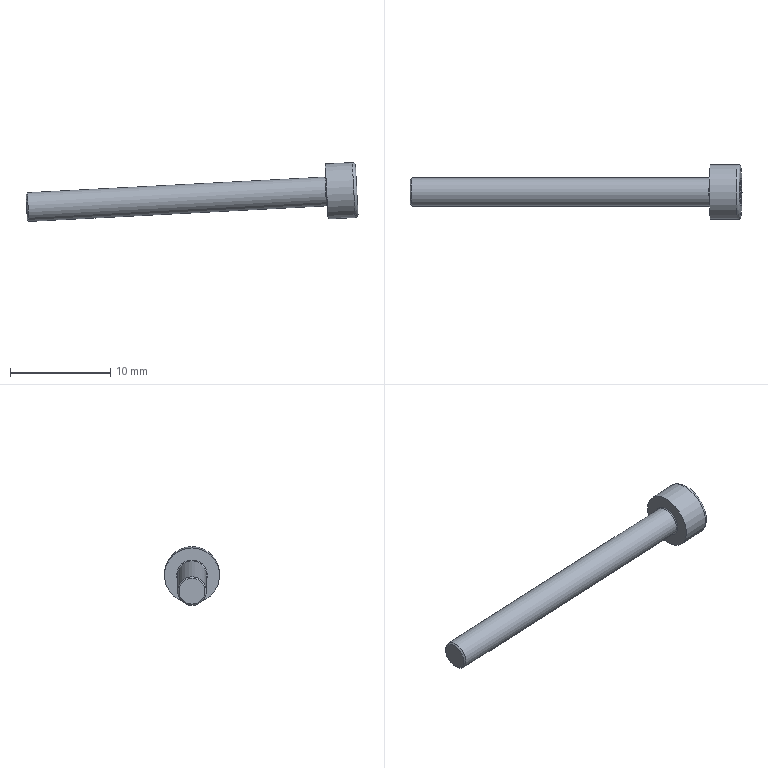Component | NX | GB-T70_1-2000_M3X30 | 1 solid | 27 faces | volume 254 mm3 | plane 15 | cone 8 | cylinder 2 | torus 2 | commonest cylinder face diameters 2.874 x1 5.5 x1